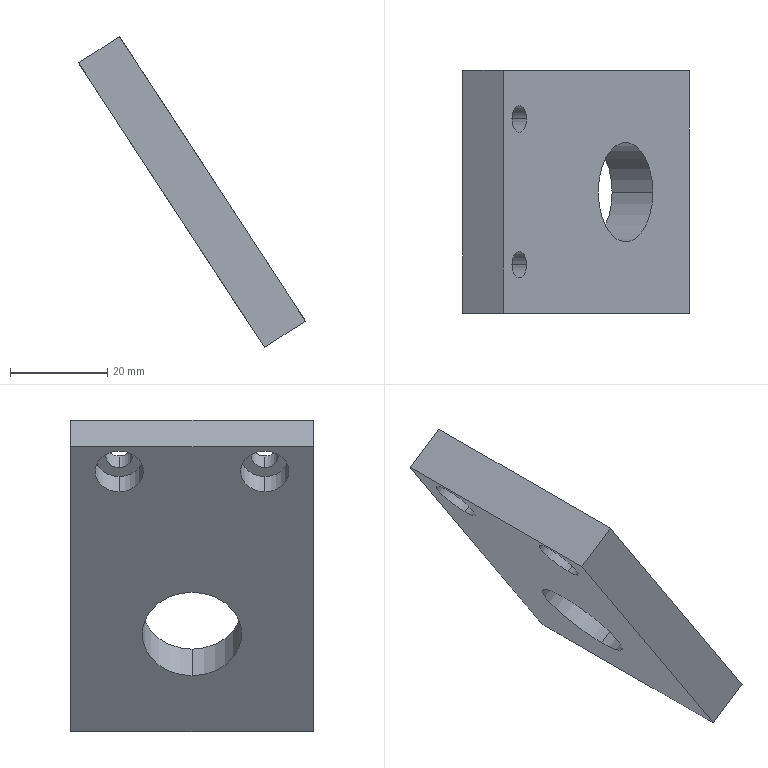Component | SolidWorks | CylinderMountingPlate01-1 | 1 solid | 18 faces | box 46.66 x 50 x 64.07 mm | volume 30600 mm3 | cylinder 10 | plane 8 | commonest cylinder face diameters 10 x4 5.5 x4 20.5 x2
build123d program:
from build123d import *

# Parameters (mm, degrees)
SKETCH1_W                                            = 70
SKETCH1_H                                            = 50
BOSS_EXTRUDE1_DEPTH                                  = 10
HOLE_SIZE_ACCORDING_TO_THE_TYPE_OF_HEXAG_D           = 5.5
HOLE_SIZE_ACCORDING_TO_THE_TYPE_OF_HEXAG_CBORE_D     = 10
HOLE_SIZE_ACCORDING_TO_THE_TYPE_OF_HEXAG_CBORE_DEPTH = 5.7
M22X1_5_TAPPED_HOLE1_D                               = 20.5
M22X1_5_TAPPED_HOLE1_DEPTH                           = 48.5
M22X1_5_TAPPED_HOLE1_TIP                             = 6.159


with BuildPart() as part:
    # Sketch1 → Boss-Extrude1 (new body)
    with BuildSketch(Plane.XY):
        Rectangle(SKETCH1_W, SKETCH1_H)
    extrude(amount=BOSS_EXTRUDE1_DEPTH)

    # Hole Size according to the type of hexag (through all)
    with Locations(Plane.XY.offset(10)):
        with Locations((-29, 15), (-29, -15)):
            CounterBoreHole(HOLE_SIZE_ACCORDING_TO_THE_TYPE_OF_HEXAG_D / 2, HOLE_SIZE_ACCORDING_TO_THE_TYPE_OF_HEXAG_CBORE_D / 2, HOLE_SIZE_ACCORDING_TO_THE_TYPE_OF_HEXAG_CBORE_DEPTH)

    # M22x1.5 Tapped Hole1
    with Locations(Plane(origin=(0, 0, 0), x_dir=(-1, 0, 0), z_dir=(0, 0, -1))):
        with Locations((-11, 0)):
            Hole(M22X1_5_TAPPED_HOLE1_D / 2, depth=M22X1_5_TAPPED_HOLE1_DEPTH)
            with Locations((0, 0, -(M22X1_5_TAPPED_HOLE1_DEPTH + M22X1_5_TAPPED_HOLE1_TIP / 2))):  # 118° drill point
                Cone(0, M22X1_5_TAPPED_HOLE1_D / 2, M22X1_5_TAPPED_HOLE1_TIP, mode=Mode.SUBTRACT)


solid = part.part

# Placed as in the assembly
solid = solid.moved(Location((-78.529, 149.546, -41.258), (180, -56.835, 0)))
STEP:
#1=COLOUR_RGB('',0.7922,0.8196,0.9333);
#2=FILL_AREA_STYLE_COLOUR('',#1);
#3=FILL_AREA_STYLE('',(#2));
#4=SURFACE_STYLE_FILL_AREA(#3);
#5=SURFACE_SIDE_STYLE('',(#4));
#6=SURFACE_STYLE_USAGE(.BOTH.,#5);
#7=PRESENTATION_STYLE_ASSIGNMENT((#6));
#8=CARTESIAN_POINT('',(-2.964,5.888,-2.54));
#9=VERTEX_POINT('',#8);
#10=CARTESIAN_POINT('',(-3.405,5.888,-1.864));
#11=VERTEX_POINT('',#10);
#12=CARTESIAN_POINT('',(-3.184,5.888,-2.202));
#13=DIRECTION('',(0.8371,0.,0.5471));
#14=DIRECTION('',(-0.5471,0.,0.8371));
#15=AXIS2_PLACEMENT_3D('',#12,#13,#14);
#16=CIRCLE('',#15,0.4035);
#17=EDGE_CURVE('',#9,#11,#16,.T.);
#18=ORIENTED_EDGE('',*,*,#17,.F.);
#19=CARTESIAN_POINT('',(-2.634,5.888,-2.325));
#20=VERTEX_POINT('',#19);
#21=CARTESIAN_POINT('',(-2.634,5.888,-2.325));
#22=DIRECTION('',(0.8371,0.,0.5471));
#23=VECTOR('',#22,39.37);
#24=LINE('',#21,#23);
#25=EDGE_CURVE('',#9,#20,#24,.T.);
#26=ORIENTED_EDGE('',*,*,#25,.T.);
#27=CARTESIAN_POINT('',(-3.076,5.888,-1.649));
#28=VERTEX_POINT('',#27);
#29=CARTESIAN_POINT('',(-2.855,5.888,-1.987));
#30=DIRECTION('',(0.8371,0.,0.5471));
#31=DIRECTION('',(-0.5471,0.,0.8371));
#32=AXIS2_PLACEMENT_3D('',#29,#30,#31);
#33=CIRCLE('',#32,0.4035);
#34=EDGE_CURVE('',#20,#28,#33,.T.);
#35=ORIENTED_EDGE('',*,*,#34,.T.);
#36=CARTESIAN_POINT('',(-3.076,5.888,-1.649));
#37=DIRECTION('',(0.8371,0.,0.5471));
#38=VECTOR('',#37,39.37);
#39=LINE('',#36,#38);
#40=EDGE_CURVE('',#11,#28,#39,.T.);
#41=ORIENTED_EDGE('',*,*,#40,.F.);
#42=EDGE_LOOP('',(#18,#26,#35,#41));
#43=FACE_OUTER_BOUND('',#42,.T.);
#44=CARTESIAN_POINT('',(-2.855,5.888,-1.987));
#45=DIRECTION('',(0.8371,0.,0.5471));
#46=DIRECTION('',(-0.5471,0.,0.8371));
#47=AXIS2_PLACEMENT_3D('',#44,#45,#46);
#48=CYLINDRICAL_SURFACE('',#47,0.4035);
#49=ADVANCED_FACE('',(#43),#48,.F.);
#50=CARTESIAN_POINT('',(-3.966,5.297,-0.5964));
#51=VERTEX_POINT('',#50);
#52=CARTESIAN_POINT('',(-3.75,5.297,-0.926));
#53=VERTEX_POINT('',#52);
#54=CARTESIAN_POINT('',(-3.858,5.297,-0.7612));
#55=DIRECTION('',(-0.8371,-0.,-0.5471));
#56=DIRECTION('',(0.5471,0.,-0.8371));
#57=AXIS2_PLACEMENT_3D('',#54,#55,#56);
#58=CIRCLE('',#57,0.1969);
#59=EDGE_CURVE('',#51,#53,#58,.T.);
#60=ORIENTED_EDGE('',*,*,#59,.F.);
#61=CARTESIAN_POINT('',(-4.154,5.297,-0.7192));
#62=VERTEX_POINT('',#61);
#63=CARTESIAN_POINT('',(-4.154,5.297,-0.7192));
#64=DIRECTION('',(-0.8371,-0.,-0.5471));
#65=VECTOR('',#64,39.37);
#66=LINE('',#63,#65);
#67=EDGE_CURVE('',#51,#62,#66,.T.);
#68=ORIENTED_EDGE('',*,*,#67,.T.);
#69=CARTESIAN_POINT('',(-3.938,5.297,-1.049));
#70=VERTEX_POINT('',#69);
#71=CARTESIAN_POINT('',(-4.046,5.297,-0.884));
#72=DIRECTION('',(-0.8371,-0.,-0.5471));
#73=DIRECTION('',(0.5471,0.,-0.8371));
#74=AXIS2_PLACEMENT_3D('',#71,#72,#73);
#75=CIRCLE('',#74,0.1969);
#76=EDGE_CURVE('',#62,#70,#75,.T.);
#77=ORIENTED_EDGE('',*,*,#76,.T.);
#78=CARTESIAN_POINT('',(-3.938,5.297,-1.049));
#79=DIRECTION('',(-0.8371,-0.,-0.5471));
#80=VECTOR('',#79,39.37);
#81=LINE('',#78,#80);
#82=EDGE_CURVE('',#53,#70,#81,.T.);
#83=ORIENTED_EDGE('',*,*,#82,.F.);
#84=EDGE_LOOP('',(#60,#68,#77,#83));
#85=FACE_OUTER_BOUND('',#84,.T.);
#86=CARTESIAN_POINT('',(-4.046,5.297,-0.884));
#87=DIRECTION('',(-0.8371,-0.,-0.5471));
#88=DIRECTION('',(0.5471,0.,-0.8371));
#89=AXIS2_PLACEMENT_3D('',#86,#87,#88);
#90=CYLINDRICAL_SURFACE('',#89,0.1969);
#91=ADVANCED_FACE('',(#85),#90,.F.);
#92=CARTESIAN_POINT('',(-3.776,5.297,-0.5779));
#93=VERTEX_POINT('',#92);
#94=CARTESIAN_POINT('',(-3.657,5.297,-0.7592));
#95=VERTEX_POINT('',#94);
#96=CARTESIAN_POINT('',(-3.716,5.297,-0.6686));
#97=DIRECTION('',(-0.8371,-0.,-0.5471));
#98=DIRECTION('',(0.5471,0.,-0.8371));
#99=AXIS2_PLACEMENT_3D('',#96,#97,#98);
#100=CIRCLE('',#99,0.1083);
#101=EDGE_CURVE('',#93,#95,#100,.T.);
#102=ORIENTED_EDGE('',*,*,#101,.F.);
#103=CARTESIAN_POINT('',(-3.917,5.297,-0.6706));
#104=VERTEX_POINT('',#103);
#105=CARTESIAN_POINT('',(-4.105,5.297,-0.7933));
#106=DIRECTION('',(-0.8371,-0.,-0.5471));
#107=VECTOR('',#106,39.37);
#108=LINE('',#105,#107);
#109=EDGE_CURVE('',#93,#104,#108,.T.);
#110=ORIENTED_EDGE('',*,*,#109,.T.);
#111=CARTESIAN_POINT('',(-3.799,5.297,-0.8518));
#112=VERTEX_POINT('',#111);
#113=CARTESIAN_POINT('',(-3.858,5.297,-0.7612));
#114=DIRECTION('',(-0.8371,-0.,-0.5471));
#115=DIRECTION('',(0.5471,0.,-0.8371));
#116=AXIS2_PLACEMENT_3D('',#113,#114,#115);
#117=CIRCLE('',#116,0.1083);
#118=EDGE_CURVE('',#104,#112,#117,.T.);
#119=ORIENTED_EDGE('',*,*,#118,.T.);
#120=CARTESIAN_POINT('',(-3.987,5.297,-0.9746));
#121=DIRECTION('',(-0.8371,-0.,-0.5471));
#122=VECTOR('',#121,39.37);
#123=LINE('',#120,#122);
#124=EDGE_CURVE('',#95,#112,#123,.T.);
#125=ORIENTED_EDGE('',*,*,#124,.F.);
#126=EDGE_LOOP('',(#102,#110,#119,#125));
#127=FACE_OUTER_BOUND('',#126,.T.);
#128=CARTESIAN_POINT('',(-4.046,5.297,-0.884));
#129=DIRECTION('',(-0.8371,-0.,-0.5471));
#130=DIRECTION('',(0.5471,0.,-0.8371));
#131=AXIS2_PLACEMENT_3D('',#128,#129,#130);
#132=CYLINDRICAL_SURFACE('',#131,0.1083);
#133=ADVANCED_FACE('',(#127),#132,.F.);
#134=CARTESIAN_POINT('',(-3.966,6.478,-0.5964));
#135=VERTEX_POINT('',#134);
#136=CARTESIAN_POINT('',(-3.75,6.478,-0.926));
#137=VERTEX_POINT('',#136);
#138=CARTESIAN_POINT('',(-3.858,6.478,-0.7612));
#139=DIRECTION('',(-0.8371,-0.,-0.5471));
#140=DIRECTION('',(0.5471,0.,-0.8371));
#141=AXIS2_PLACEMENT_3D('',#138,#139,#140);
#142=CIRCLE('',#141,0.1969);
#143=EDGE_CURVE('',#135,#137,#142,.T.);
#144=ORIENTED_EDGE('',*,*,#143,.F.);
#145=CARTESIAN_POINT('',(-4.154,6.478,-0.7192));
#146=VERTEX_POINT('',#145);
#147=CARTESIAN_POINT('',(-4.154,6.478,-0.7192));
#148=DIRECTION('',(-0.8371,-0.,-0.5471));
#149=VECTOR('',#148,39.37);
#150=LINE('',#147,#149);
#151=EDGE_CURVE('',#135,#146,#150,.T.);
#152=ORIENTED_EDGE('',*,*,#151,.T.);
#153=CARTESIAN_POINT('',(-3.938,6.478,-1.049));
#154=VERTEX_POINT('',#153);
#155=CARTESIAN_POINT('',(-4.046,6.478,-0.884));
#156=DIRECTION('',(-0.8371,-0.,-0.5471));
#157=DIRECTION('',(0.5471,0.,-0.8371));
#158=AXIS2_PLACEMENT_3D('',#155,#156,#157);
#159=CIRCLE('',#158,0.1969);
#160=EDGE_CURVE('',#146,#154,#159,.T.);
#161=ORIENTED_EDGE('',*,*,#160,.T.);
#162=CARTESIAN_POINT('',(-3.938,6.478,-1.049));
#163=DIRECTION('',(-0.8371,-0.,-0.5471));
#164=VECTOR('',#163,39.37);
#165=LINE('',#162,#164);
#166=EDGE_CURVE('',#137,#154,#165,.T.);
#167=ORIENTED_EDGE('',*,*,#166,.F.);
#168=EDGE_LOOP('',(#144,#152,#161,#167));
#169=FACE_OUTER_BOUND('',#168,.T.);
#170=CARTESIAN_POINT('',(-4.046,6.478,-0.884));
#171=DIRECTION('',(-0.8371,-0.,-0.5471));
#172=DIRECTION('',(0.5471,0.,-0.8371));
#173=AXIS2_PLACEMENT_3D('',#170,#171,#172);
#174=CYLINDRICAL_SURFACE('',#173,0.1969);
#175=ADVANCED_FACE('',(#169),#174,.F.);
#176=CARTESIAN_POINT('',(-3.776,6.478,-0.5779));
#177=VERTEX_POINT('',#176);
#178=CARTESIAN_POINT('',(-3.657,6.478,-0.7592));
#179=VERTEX_POINT('',#178);
#180=CARTESIAN_POINT('',(-3.716,6.478,-0.6686));
#181=DIRECTION('',(-0.8371,-0.,-0.5471));
#182=DIRECTION('',(0.5471,0.,-0.8371));
#183=AXIS2_PLACEMENT_3D('',#180,#181,#182);
#184=CIRCLE('',#183,0.1083);
#185=EDGE_CURVE('',#177,#179,#184,.T.);
#186=ORIENTED_EDGE('',*,*,#185,.F.);
#187=CARTESIAN_POINT('',(-3.917,6.478,-0.6706));
#188=VERTEX_POINT('',#187);
#189=CARTESIAN_POINT('',(-4.105,6.478,-0.7933));
#190=DIRECTION('',(-0.8371,-0.,-0.5471));
#191=VECTOR('',#190,39.37);
#192=LINE('',#189,#191);
#193=EDGE_CURVE('',#177,#188,#192,.T.);
#194=ORIENTED_EDGE('',*,*,#193,.T.);
#195=CARTESIAN_POINT('',(-3.799,6.478,-0.8518));
#196=VERTEX_POINT('',#195);
#197=CARTESIAN_POINT('',(-3.858,6.478,-0.7612));
#198=DIRECTION('',(-0.8371,-0.,-0.5471));
#199=DIRECTION('',(0.5471,0.,-0.8371));
#200=AXIS2_PLACEMENT_3D('',#197,#198,#199);
#201=CIRCLE('',#200,0.1083);
#202=EDGE_CURVE('',#188,#196,#201,.T.);
#203=ORIENTED_EDGE('',*,*,#202,.T.);
#204=CARTESIAN_POINT('',(-3.987,6.478,-0.9746));
#205=DIRECTION('',(-0.8371,-0.,-0.5471));
#206=VECTOR('',#205,39.37);
#207=LINE('',#204,#206);
#208=EDGE_CURVE('',#179,#196,#207,.T.);
#209=ORIENTED_EDGE('',*,*,#208,.F.);
#210=EDGE_LOOP('',(#186,#194,#203,#209));
#211=FACE_OUTER_BOUND('',#210,.T.);
#212=CARTESIAN_POINT('',(-4.046,6.478,-0.884));
#213=DIRECTION('',(-0.8371,-0.,-0.5471));
#214=DIRECTION('',(0.5471,0.,-0.8371));
#215=AXIS2_PLACEMENT_3D('',#212,#213,#214);
#216=CYLINDRICAL_SURFACE('',#215,0.1083);
#217=ADVANCED_FACE('',(#211),#216,.F.);
#218=CARTESIAN_POINT('',(-2.338,6.872,-2.778));
#219=VERTEX_POINT('',#218);
#220=CARTESIAN_POINT('',(-2.338,4.903,-2.778));
#221=VERTEX_POINT('',#220);
#222=CARTESIAN_POINT('',(-2.338,6.872,-2.778));
#223=DIRECTION('',(-0.,-1.,0.));
#224=VECTOR('',#223,39.37);
#225=LINE('',#222,#224);
#226=EDGE_CURVE('',#219,#221,#225,.T.);
#227=ORIENTED_EDGE('',*,*,#226,.T.);
#228=CARTESIAN_POINT('',(-2.667,4.903,-2.993));
#229=VERTEX_POINT('',#228);
#230=CARTESIAN_POINT('',(-2.667,4.903,-2.993));
#231=DIRECTION('',(0.8371,0.,0.5471));
#232=VECTOR('',#231,39.37);
#233=LINE('',#230,#232);
#234=EDGE_CURVE('',#229,#221,#233,.T.);
#235=ORIENTED_EDGE('',*,*,#234,.F.);
#236=CARTESIAN_POINT('',(-2.667,6.872,-2.993));
#237=VERTEX_POINT('',#236);
#238=CARTESIAN_POINT('',(-2.667,6.872,-2.993));
#239=DIRECTION('',(-0.,-1.,0.));
#240=VECTOR('',#239,39.37);
#241=LINE('',#238,#240);
#242=EDGE_CURVE('',#237,#229,#241,.T.);
#243=ORIENTED_EDGE('',*,*,#242,.F.);
#244=CARTESIAN_POINT('',(-2.667,6.872,-2.993));
#245=DIRECTION('',(0.8371,0.,0.5471));
#246=VECTOR('',#245,39.37);
#247=LINE('',#244,#246);
#248=EDGE_CURVE('',#237,#219,#247,.T.);
#249=ORIENTED_EDGE('',*,*,#248,.T.);
#250=EDGE_LOOP('',(#227,#235,#243,#249));
#251=FACE_OUTER_BOUND('',#250,.T.);
#252=CARTESIAN_POINT('',(-2.667,6.872,-2.993));
#253=DIRECTION('',(-0.5471,0.,0.8371));
#254=DIRECTION('',(-0.8371,-0.,-0.5471));
#255=AXIS2_PLACEMENT_3D('',#252,#253,#254);
#256=PLANE('',#255);
#257=ADVANCED_FACE('',(#251),#256,.F.);
#258=CARTESIAN_POINT('',(-3.845,4.903,-0.4708));
#259=VERTEX_POINT('',#258);
#260=CARTESIAN_POINT('',(-3.845,4.903,-0.4708));
#261=DIRECTION('',(-0.5471,0.,0.8371));
#262=VECTOR('',#261,39.37);
#263=LINE('',#260,#262);
#264=EDGE_CURVE('',#221,#259,#263,.T.);
#265=ORIENTED_EDGE('',*,*,#264,.T.);
#266=CARTESIAN_POINT('',(-4.175,4.903,-0.6862));
#267=VERTEX_POINT('',#266);
#268=CARTESIAN_POINT('',(-4.175,4.903,-0.6862));
#269=DIRECTION('',(0.8371,0.,0.5471));
#270=VECTOR('',#269,39.37);
#271=LINE('',#268,#270);
#272=EDGE_CURVE('',#267,#259,#271,.T.);
#273=ORIENTED_EDGE('',*,*,#272,.F.);
#274=CARTESIAN_POINT('',(-4.175,4.903,-0.6862));
#275=DIRECTION('',(-0.5471,0.,0.8371));
#276=VECTOR('',#275,39.37);
#277=LINE('',#274,#276);
#278=EDGE_CURVE('',#229,#267,#277,.T.);
#279=ORIENTED_EDGE('',*,*,#278,.F.);
#280=ORIENTED_EDGE('',*,*,#234,.T.);
#281=EDGE_LOOP('',(#265,#273,#279,#280));
#282=FACE_OUTER_BOUND('',#281,.T.);
#283=CARTESIAN_POINT('',(-4.175,4.903,-0.6862));
#284=DIRECTION('',(0.,1.,-0.));
#285=DIRECTION('',(0.8371,0.,0.5471));
#286=AXIS2_PLACEMENT_3D('',#283,#284,#285);
#287=PLANE('',#286);
#288=ADVANCED_FACE('',(#282),#287,.F.);
#289=CARTESIAN_POINT('',(-3.845,6.872,-0.4708));
#290=VERTEX_POINT('',#289);
#291=CARTESIAN_POINT('',(-3.845,6.872,-0.4708));
#292=DIRECTION('',(0.,1.,-0.));
#293=VECTOR('',#292,39.37);
#294=LINE('',#291,#293);
#295=EDGE_CURVE('',#259,#290,#294,.T.);
#296=ORIENTED_EDGE('',*,*,#295,.T.);
#297=CARTESIAN_POINT('',(-4.175,6.872,-0.6862));
#298=VERTEX_POINT('',#297);
#299=CARTESIAN_POINT('',(-4.175,6.872,-0.6862));
#300=DIRECTION('',(0.8371,0.,0.5471));
#301=VECTOR('',#300,39.37);
#302=LINE('',#299,#301);
#303=EDGE_CURVE('',#298,#290,#302,.T.);
#304=ORIENTED_EDGE('',*,*,#303,.F.);
#305=CARTESIAN_POINT('',(-4.175,6.872,-0.6862));
#306=DIRECTION('',(0.,1.,-0.));
#307=VECTOR('',#306,39.37);
#308=LINE('',#305,#307);
#309=EDGE_CURVE('',#267,#298,#308,.T.);
#310=ORIENTED_EDGE('',*,*,#309,.F.);
#311=ORIENTED_EDGE('',*,*,#272,.T.);
#312=EDGE_LOOP('',(#296,#304,#310,#311));
#313=FACE_OUTER_BOUND('',#312,.T.);
#314=CARTESIAN_POINT('',(-4.175,6.872,-0.6862));
#315=DIRECTION('',(0.5471,-0.,-0.8371));
#316=DIRECTION('',(0.8371,0.,0.5471));
#317=AXIS2_PLACEMENT_3D('',#314,#315,#316);
#318=PLANE('',#317);
#319=ADVANCED_FACE('',(#313),#318,.F.);
#320=CARTESIAN_POINT('',(-3.845,6.872,-0.4708));
#321=DIRECTION('',(0.5471,-0.,-0.8371));
#322=VECTOR('',#321,39.37);
#323=LINE('',#320,#322);
#324=EDGE_CURVE('',#290,#219,#323,.T.);
#325=ORIENTED_EDGE('',*,*,#324,.T.);
#326=ORIENTED_EDGE('',*,*,#248,.F.);
#327=CARTESIAN_POINT('',(-4.175,6.872,-0.6862));
#328=DIRECTION('',(0.5471,-0.,-0.8371));
#329=VECTOR('',#328,39.37);
#330=LINE('',#327,#329);
#331=EDGE_CURVE('',#298,#237,#330,.T.);
#332=ORIENTED_EDGE('',*,*,#331,.F.);
#333=ORIENTED_EDGE('',*,*,#303,.T.);
#334=EDGE_LOOP('',(#325,#326,#332,#333));
#335=FACE_OUTER_BOUND('',#334,.T.);
#336=CARTESIAN_POINT('',(-4.175,6.872,-0.6862));
#337=DIRECTION('',(-0.,-1.,0.));
#338=DIRECTION('',(-0.8371,-0.,-0.5471));
#339=AXIS2_PLACEMENT_3D('',#336,#337,#338);
#340=PLANE('',#339);
#341=ADVANCED_FACE('',(#335),#340,.F.);
#342=CARTESIAN_POINT('',(-3.184,5.888,-2.202));
#343=DIRECTION('',(0.8371,0.,0.5471));
#344=DIRECTION('',(-0.5471,0.,0.8371));
#345=AXIS2_PLACEMENT_3D('',#342,#343,#344);
#346=CIRCLE('',#345,0.4035);
#347=EDGE_CURVE('',#11,#9,#346,.T.);
#348=ORIENTED_EDGE('',*,*,#347,.T.);
#349=ORIENTED_EDGE('',*,*,#17,.T.);
#350=EDGE_LOOP('',(#348,#349));
#351=FACE_BOUND('',#350,.T.);
#352=CARTESIAN_POINT('',(-4.046,5.297,-0.884));
#353=DIRECTION('',(-0.8371,-0.,-0.5471));
#354=DIRECTION('',(0.5471,0.,-0.8371));
#355=AXIS2_PLACEMENT_3D('',#352,#353,#354);
#356=CIRCLE('',#355,0.1969);
#357=EDGE_CURVE('',#70,#62,#356,.T.);
#358=ORIENTED_EDGE('',*,*,#357,.F.);
#359=ORIENTED_EDGE('',*,*,#76,.F.);
#360=EDGE_LOOP('',(#358,#359));
#361=FACE_BOUND('',#360,.T.);
#362=CARTESIAN_POINT('',(-4.046,6.478,-0.884));
#363=DIRECTION('',(-0.8371,-0.,-0.5471));
#364=DIRECTION('',(0.5471,0.,-0.8371));
#365=AXIS2_PLACEMENT_3D('',#362,#363,#364);
#366=CIRCLE('',#365,0.1969);
#367=EDGE_CURVE('',#154,#146,#366,.T.);
#368=ORIENTED_EDGE('',*,*,#367,.F.);
#369=ORIENTED_EDGE('',*,*,#160,.F.);
#370=EDGE_LOOP('',(#368,#369));
#371=FACE_BOUND('',#370,.T.);
#372=ORIENTED_EDGE('',*,*,#242,.T.);
#373=ORIENTED_EDGE('',*,*,#278,.T.);
#374=ORIENTED_EDGE('',*,*,#309,.T.);
#375=ORIENTED_EDGE('',*,*,#331,.T.);
#376=EDGE_LOOP('',(#372,#373,#374,#375));
#377=FACE_OUTER_BOUND('',#376,.T.);
#378=CARTESIAN_POINT('',(-3.421,5.888,-1.84));
#379=DIRECTION('',(0.8371,0.,0.5471));
#380=DIRECTION('',(-0.5471,0.,0.8371));
#381=AXIS2_PLACEMENT_3D('',#378,#379,#380);
#382=PLANE('',#381);
#383=ADVANCED_FACE('',(#351,#361,#371,#377),#382,.F.);
#384=CARTESIAN_POINT('',(-2.855,5.888,-1.987));
#385=DIRECTION('',(0.8371,0.,0.5471));
#386=DIRECTION('',(-0.5471,0.,0.8371));
#387=AXIS2_PLACEMENT_3D('',#384,#385,#386);
#388=CIRCLE('',#387,0.4035);
#389=EDGE_CURVE('',#28,#20,#388,.T.);
#390=ORIENTED_EDGE('',*,*,#389,.F.);
#391=ORIENTED_EDGE('',*,*,#34,.F.);
#392=EDGE_LOOP('',(#390,#391));
#393=FACE_BOUND('',#392,.T.);
#394=CARTESIAN_POINT('',(-3.716,5.297,-0.6686));
#395=DIRECTION('',(-0.8371,-0.,-0.5471));
#396=DIRECTION('',(0.5471,0.,-0.8371));
#397=AXIS2_PLACEMENT_3D('',#394,#395,#396);
#398=CIRCLE('',#397,0.1083);
#399=EDGE_CURVE('',#95,#93,#398,.T.);
#400=ORIENTED_EDGE('',*,*,#399,.T.);
#401=ORIENTED_EDGE('',*,*,#101,.T.);
#402=EDGE_LOOP('',(#400,#401));
#403=FACE_BOUND('',#402,.T.);
#404=CARTESIAN_POINT('',(-3.716,6.478,-0.6686));
#405=DIRECTION('',(-0.8371,-0.,-0.5471));
#406=DIRECTION('',(0.5471,0.,-0.8371));
#407=AXIS2_PLACEMENT_3D('',#404,#405,#406);
#408=CIRCLE('',#407,0.1083);
#409=EDGE_CURVE('',#179,#177,#408,.T.);
#410=ORIENTED_EDGE('',*,*,#409,.T.);
#411=ORIENTED_EDGE('',*,*,#185,.T.);
#412=EDGE_LOOP('',(#410,#411));
#413=FACE_BOUND('',#412,.T.);
#414=ORIENTED_EDGE('',*,*,#226,.F.);
#415=ORIENTED_EDGE('',*,*,#324,.F.);
#416=ORIENTED_EDGE('',*,*,#295,.F.);
#417=ORIENTED_EDGE('',*,*,#264,.F.);
#418=EDGE_LOOP('',(#414,#415,#416,#417));
#419=FACE_OUTER_BOUND('',#418,.T.);
#420=CARTESIAN_POINT('',(-3.092,5.888,-1.624));
#421=DIRECTION('',(0.8371,0.,0.5471));
#422=DIRECTION('',(-0.5471,0.,0.8371));
#423=AXIS2_PLACEMENT_3D('',#420,#421,#422);
#424=PLANE('',#423);
#425=ADVANCED_FACE('',(#393,#403,#413,#419),#424,.T.);
#426=ORIENTED_EDGE('',*,*,#193,.F.);
#427=ORIENTED_EDGE('',*,*,#409,.F.);
#428=ORIENTED_EDGE('',*,*,#208,.T.);
#429=CARTESIAN_POINT('',(-3.858,6.478,-0.7612));
#430=DIRECTION('',(-0.8371,-0.,-0.5471));
#431=DIRECTION('',(0.5471,0.,-0.8371));
#432=AXIS2_PLACEMENT_3D('',#429,#430,#431);
#433=CIRCLE('',#432,0.1083);
#434=EDGE_CURVE('',#196,#188,#433,.T.);
#435=ORIENTED_EDGE('',*,*,#434,.T.);
#436=EDGE_LOOP('',(#426,#427,#428,#435));
#437=FACE_OUTER_BOUND('',#436,.T.);
#438=CARTESIAN_POINT('',(-4.046,6.478,-0.884));
#439=DIRECTION('',(-0.8371,-0.,-0.5471));
#440=DIRECTION('',(0.5471,0.,-0.8371));
#441=AXIS2_PLACEMENT_3D('',#438,#439,#440);
#442=CYLINDRICAL_SURFACE('',#441,0.1083);
#443=ADVANCED_FACE('',(#437),#442,.F.);
#444=ORIENTED_EDGE('',*,*,#434,.F.);
#445=ORIENTED_EDGE('',*,*,#202,.F.);
#446=EDGE_LOOP('',(#444,#445));
#447=FACE_BOUND('',#446,.T.);
#448=CARTESIAN_POINT('',(-3.858,6.478,-0.7612));
#449=DIRECTION('',(-0.8371,-0.,-0.5471));
#450=DIRECTION('',(0.5471,0.,-0.8371));
#451=AXIS2_PLACEMENT_3D('',#448,#449,#450);
#452=CIRCLE('',#451,0.1969);
#453=EDGE_CURVE('',#137,#135,#452,.T.);
#454=ORIENTED_EDGE('',*,*,#453,.T.);
#455=ORIENTED_EDGE('',*,*,#143,.T.);
#456=EDGE_LOOP('',(#454,#455));
#457=FACE_OUTER_BOUND('',#456,.T.);
#458=CARTESIAN_POINT('',(-3.799,6.478,-0.8518));
#459=DIRECTION('',(0.8371,0.,0.5471));
#460=DIRECTION('',(-0.5471,0.,0.8371));
#461=AXIS2_PLACEMENT_3D('',#458,#459,#460);
#462=PLANE('',#461);
#463=ADVANCED_FACE('',(#447,#457),#462,.F.);
#464=ORIENTED_EDGE('',*,*,#151,.F.);
#465=ORIENTED_EDGE('',*,*,#453,.F.);
#466=ORIENTED_EDGE('',*,*,#166,.T.);
#467=ORIENTED_EDGE('',*,*,#367,.T.);
#468=EDGE_LOOP('',(#464,#465,#466,#467));
#469=FACE_OUTER_BOUND('',#468,.T.);
#470=CARTESIAN_POINT('',(-4.046,6.478,-0.884));
#471=DIRECTION('',(-0.8371,-0.,-0.5471));
#472=DIRECTION('',(0.5471,0.,-0.8371));
#473=AXIS2_PLACEMENT_3D('',#470,#471,#472);
#474=CYLINDRICAL_SURFACE('',#473,0.1969);
#475=ADVANCED_FACE('',(#469),#474,.F.);
#476=ORIENTED_EDGE('',*,*,#109,.F.);
#477=ORIENTED_EDGE('',*,*,#399,.F.);
#478=ORIENTED_EDGE('',*,*,#124,.T.);
#479=CARTESIAN_POINT('',(-3.858,5.297,-0.7612));
#480=DIRECTION('',(-0.8371,-0.,-0.5471));
#481=DIRECTION('',(0.5471,0.,-0.8371));
#482=AXIS2_PLACEMENT_3D('',#479,#480,#481);
#483=CIRCLE('',#482,0.1083);
#484=EDGE_CURVE('',#112,#104,#483,.T.);
#485=ORIENTED_EDGE('',*,*,#484,.T.);
#486=EDGE_LOOP('',(#476,#477,#478,#485));
#487=FACE_OUTER_BOUND('',#486,.T.);
#488=CARTESIAN_POINT('',(-4.046,5.297,-0.884));
#489=DIRECTION('',(-0.8371,-0.,-0.5471));
#490=DIRECTION('',(0.5471,0.,-0.8371));
#491=AXIS2_PLACEMENT_3D('',#488,#489,#490);
#492=CYLINDRICAL_SURFACE('',#491,0.1083);
#493=ADVANCED_FACE('',(#487),#492,.F.);
#494=ORIENTED_EDGE('',*,*,#484,.F.);
#495=ORIENTED_EDGE('',*,*,#118,.F.);
#496=EDGE_LOOP('',(#494,#495));
#497=FACE_BOUND('',#496,.T.);
#498=CARTESIAN_POINT('',(-3.858,5.297,-0.7612));
#499=DIRECTION('',(-0.8371,-0.,-0.5471));
#500=DIRECTION('',(0.5471,0.,-0.8371));
#501=AXIS2_PLACEMENT_3D('',#498,#499,#500);
#502=CIRCLE('',#501,0.1969);
#503=EDGE_CURVE('',#53,#51,#502,.T.);
#504=ORIENTED_EDGE('',*,*,#503,.T.);
#505=ORIENTED_EDGE('',*,*,#59,.T.);
#506=EDGE_LOOP('',(#504,#505));
#507=FACE_OUTER_BOUND('',#506,.T.);
#508=CARTESIAN_POINT('',(-3.799,5.297,-0.8518));
#509=DIRECTION('',(0.8371,0.,0.5471));
#510=DIRECTION('',(-0.5471,0.,0.8371));
#511=AXIS2_PLACEMENT_3D('',#508,#509,#510);
#512=PLANE('',#511);
#513=ADVANCED_FACE('',(#497,#507),#512,.F.);
#514=ORIENTED_EDGE('',*,*,#67,.F.);
#515=ORIENTED_EDGE('',*,*,#503,.F.);
#516=ORIENTED_EDGE('',*,*,#82,.T.);
#517=ORIENTED_EDGE('',*,*,#357,.T.);
#518=EDGE_LOOP('',(#514,#515,#516,#517));
#519=FACE_OUTER_BOUND('',#518,.T.);
#520=CARTESIAN_POINT('',(-4.046,5.297,-0.884));
#521=DIRECTION('',(-0.8371,-0.,-0.5471));
#522=DIRECTION('',(0.5471,0.,-0.8371));
#523=AXIS2_PLACEMENT_3D('',#520,#521,#522);
#524=CYLINDRICAL_SURFACE('',#523,0.1969);
#525=ADVANCED_FACE('',(#519),#524,.F.);
#526=ORIENTED_EDGE('',*,*,#25,.F.);
#527=ORIENTED_EDGE('',*,*,#347,.F.);
#528=ORIENTED_EDGE('',*,*,#40,.T.);
#529=ORIENTED_EDGE('',*,*,#389,.T.);
#530=EDGE_LOOP('',(#526,#527,#528,#529));
#531=FACE_OUTER_BOUND('',#530,.T.);
#532=CARTESIAN_POINT('',(-2.855,5.888,-1.987));
#533=DIRECTION('',(0.8371,0.,0.5471));
#534=DIRECTION('',(-0.5471,0.,0.8371));
#535=AXIS2_PLACEMENT_3D('',#532,#533,#534);
#536=CYLINDRICAL_SURFACE('',#535,0.4035);
#537=ADVANCED_FACE('',(#531),#536,.F.);
#538=CLOSED_SHELL('',(#49,#91,#133,#175,#217,#257,#288,#319,#341,#383,#425,#443,#463,#475,#493,#513,#525,#537));
#539=MANIFOLD_SOLID_BREP('',#538);
#540=STYLED_ITEM('',(#7),#539);
#541=PRESENTATION_LAYER_ASSIGNMENT('','',(#540));
#542=CARTESIAN_POINT('',(0.,0.,0.));
#543=DIRECTION('',(0.,0.,1.));
#544=DIRECTION('',(1.,0.,0.));
#545=AXIS2_PLACEMENT_3D('',#542,#543,#544);
#546=(LENGTH_UNIT()NAMED_UNIT(*)SI_UNIT($,.METRE.));
#547=LENGTH_MEASURE_WITH_UNIT(LENGTH_MEASURE(0.0254),#546);
#548=DIMENSIONAL_EXPONENTS(1.,0.,0.,0.,0.,0.,0.);
#549=(CONVERSION_BASED_UNIT('',#547)LENGTH_UNIT()NAMED_UNIT(#548));
#550=UNCERTAINTY_MEASURE_WITH_UNIT(LENGTH_MEASURE(0.00001),#549,'','');
#551=(NAMED_UNIT(*)PLANE_ANGLE_UNIT()SI_UNIT($,.RADIAN.));
#552=(NAMED_UNIT(*)SI_UNIT($,.STERADIAN.)SOLID_ANGLE_UNIT());
#553=(GEOMETRIC_REPRESENTATION_CONTEXT(3)GLOBAL_UNCERTAINTY_ASSIGNED_CONTEXT((#550))GLOBAL_UNIT_ASSIGNED_CONTEXT((#549,#551,#552))REPRESENTATION_CONTEXT('',''));
#554=ADVANCED_BREP_SHAPE_REPRESENTATION('',(#539,#545),#553);
#555=(LENGTH_UNIT()NAMED_UNIT(*)SI_UNIT($,.METRE.));
#556=LENGTH_MEASURE_WITH_UNIT(LENGTH_MEASURE(0.0254),#555);
#557=DIMENSIONAL_EXPONENTS(1.,0.,0.,0.,0.,0.,0.);
#558=(CONVERSION_BASED_UNIT('',#556)LENGTH_UNIT()NAMED_UNIT(#557));
#559=UNCERTAINTY_MEASURE_WITH_UNIT(LENGTH_MEASURE(0.00001),#558,'','');
#560=(NAMED_UNIT(*)PLANE_ANGLE_UNIT()SI_UNIT($,.RADIAN.));
#561=(NAMED_UNIT(*)SI_UNIT($,.STERADIAN.)SOLID_ANGLE_UNIT());
#562=(GEOMETRIC_REPRESENTATION_CONTEXT(3)GLOBAL_UNCERTAINTY_ASSIGNED_CONTEXT((#559))GLOBAL_UNIT_ASSIGNED_CONTEXT((#558,#560,#561))REPRESENTATION_CONTEXT('',''));
#563=MECHANICAL_DESIGN_GEOMETRIC_PRESENTATION_REPRESENTATION('',(#540),#562);